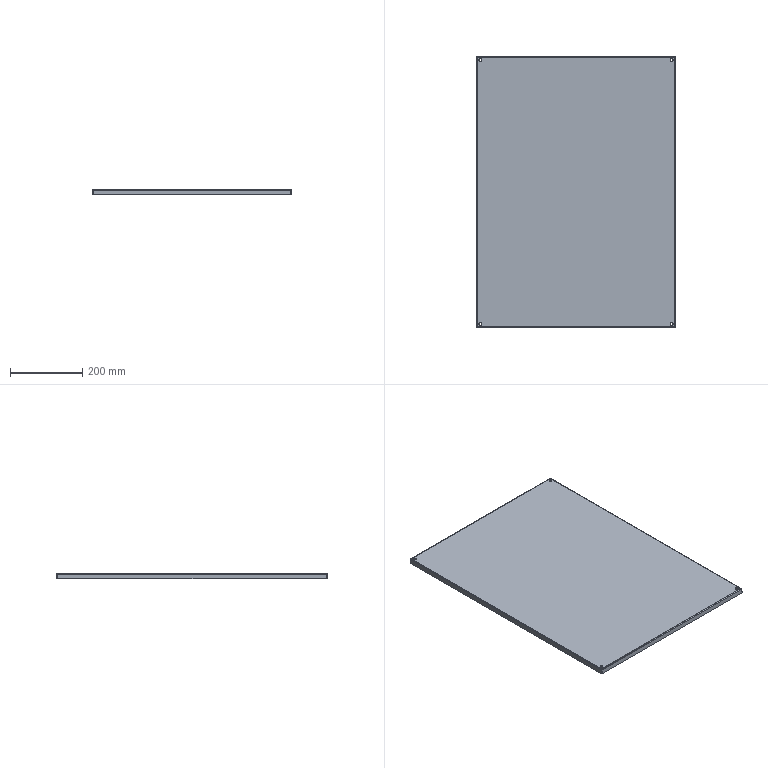Component | SolidWorks | MountingPlate-1 | 1 solid | 50 faces | volume 889532 mm3 | plane 34 | cylinder 16 | commonest cylinder face diameters 8 x8 4.2 x4 0.2 x4